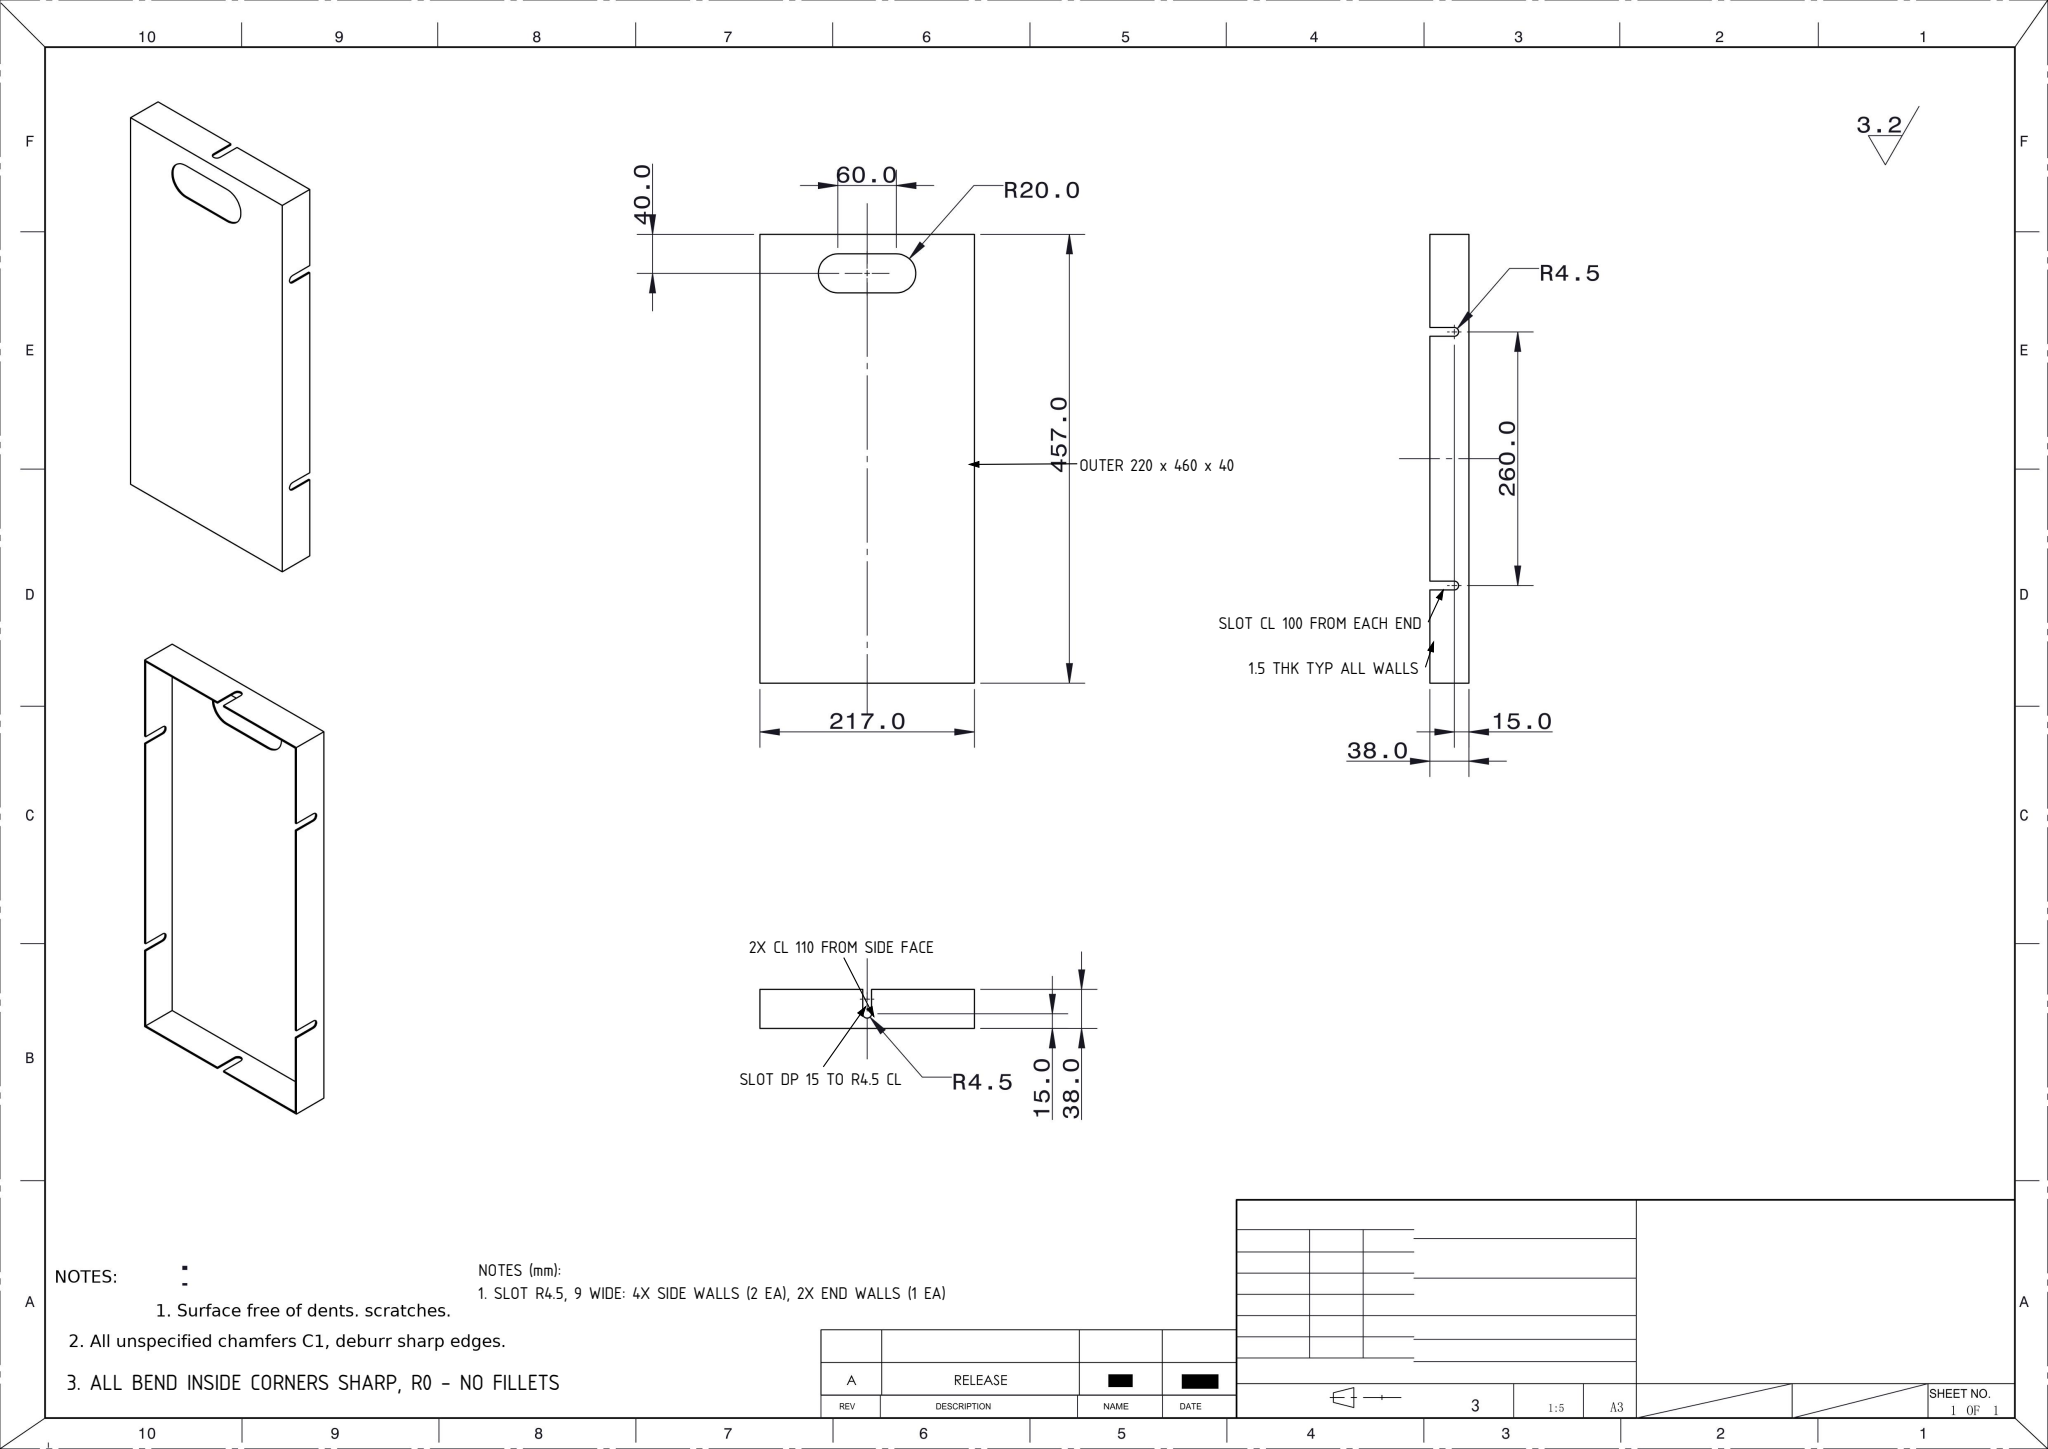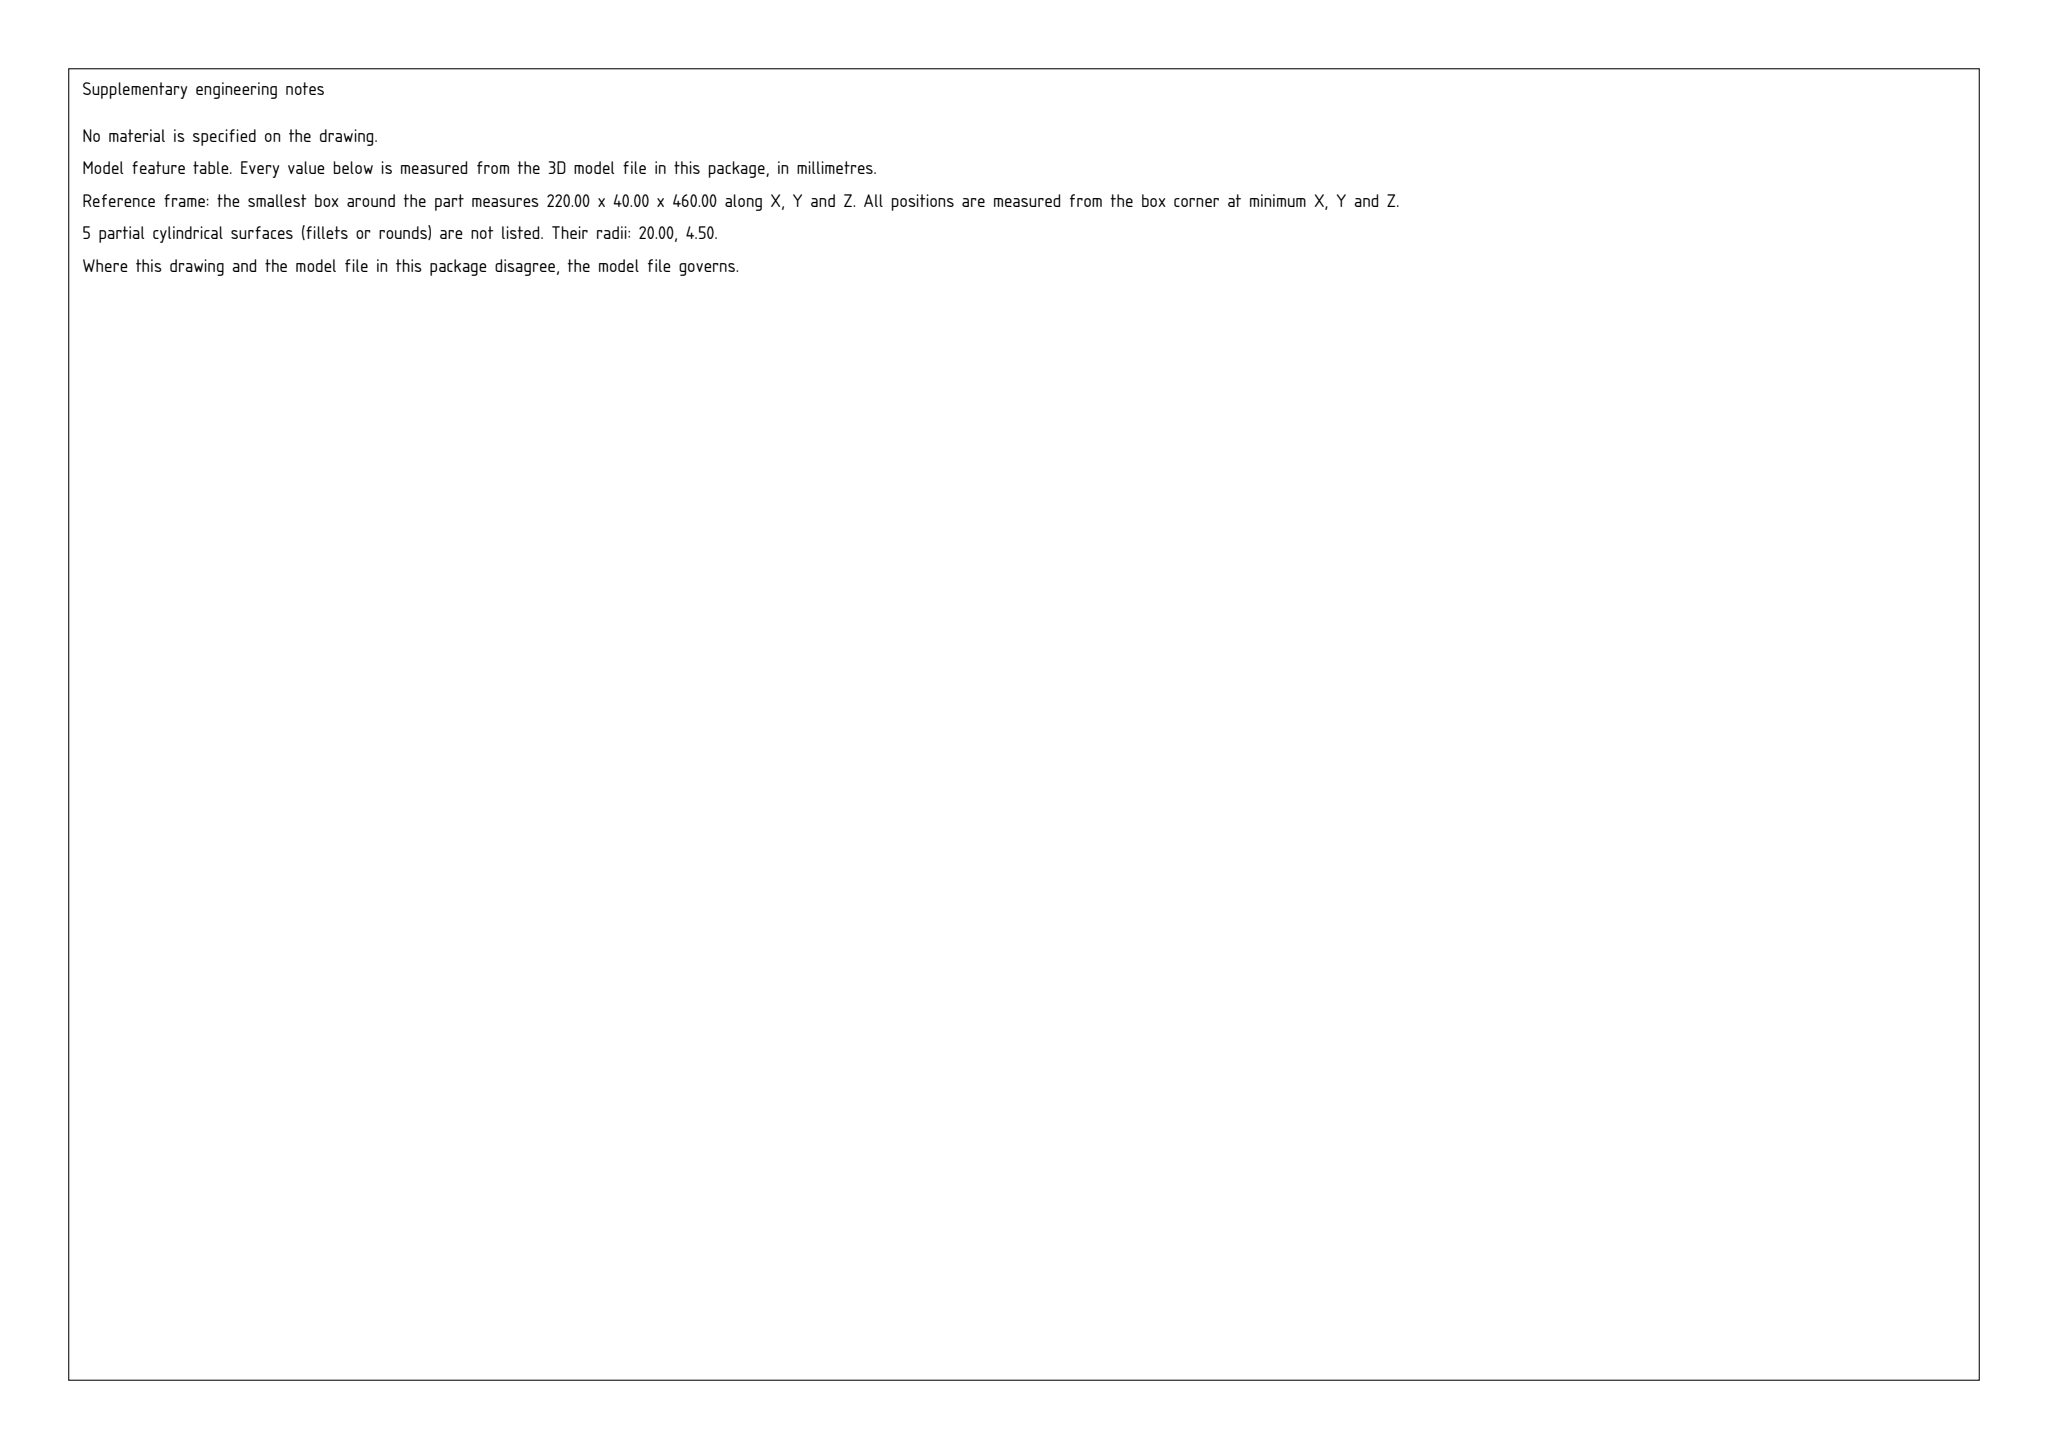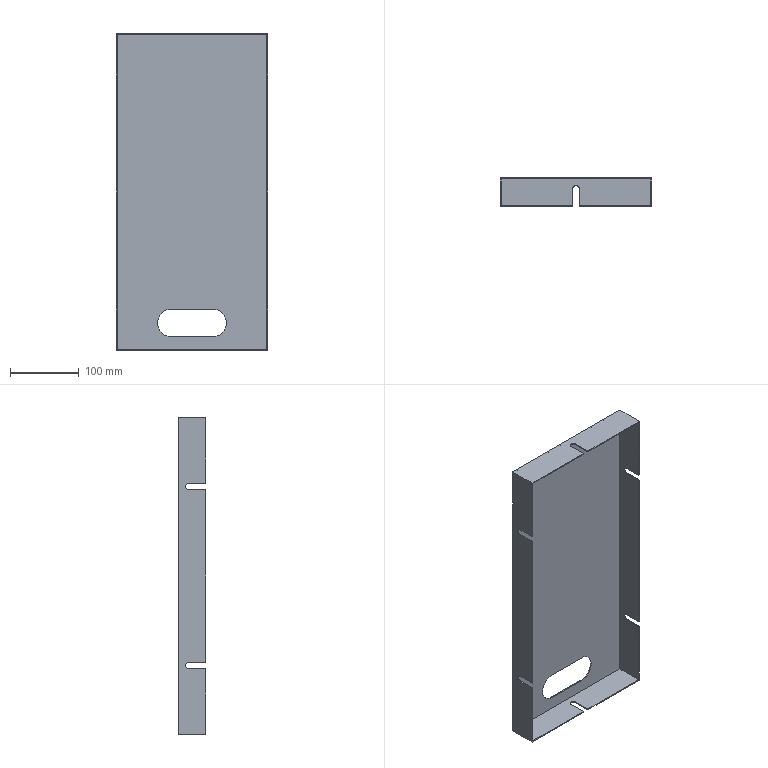Part | SolidWorks | mm | 1 solid | 38 faces | box 220 x 40 x 460 mm | volume 222197 mm3 | plane 30 | cylinder 8 | commonest cylinder face diameters 9 x6 40 x2
Drawing notes:
SHEET THK 1.5 TYP ALL WALLS, FORMED TRAY | from the solid: Planes x=0/1.5, x=218.5/220, z=0/1.5, z=458.5/460, y=38.5/40 give 1.5 wall
OVERALL OUTER ENVELOPE 220 x 460 x 40 (INNER 217 x 457) | from the solid: bbox_xyz 220.0 x 40.0 x 460.0; inner = 220-2x1.5, 460-2x1.5
ALL BEND INSIDE CORNERS SHARP, R0 - NO FILLETS | from the solid: fillet_radii: [] (empty), no cones/rounds at wall junctions
SLOT R4.5, 9 WIDE: 4X SIDE WALLS (2 EA), 2X END WALLS (1 EA) | from the solid: Ø9 x-axis cyl at z=100 (2) and z=360 (2); Ø9 z-axis cyl at x=110 (2)
SIDE WALL SLOT CL 100 FROM EACH END, 260 APART, TYP BOTH SIDES | from the solid: Ø9 x-axis cyl pos z=100 and z=360; 360-100=260; count 2 each
END WALL SLOT CL 110 FROM SIDE FACE, SYM ABOUT CL, 2X | from the solid: Ø9 z-axis cyl at x=110, count 2; bbox x=220 so 110 = CL
SLOT DEPTH 15.0 TO R4.5 CL FROM OPEN EDGE, THRU 1.5 WALL | from the solid: Ø9 cyl at y=25, wall y 0-40, length 1.5; 40-25=15
build123d program:
from build123d import *

# Parameters (mm, degrees)
SKETCH1_W           = 220
SKETCH1_H           = 460
BOSS_EXTRUDE1_DEPTH = 40
SHELL1_T            = -1.5
CUT_EXTRUDE1_DEPTH  = 1609.843
CUT_EXTRUDE2_DEPTH  = 1612.854
CUT_EXTRUDE3_DEPTH  = 502.897


with BuildPart() as part:
    # Sketch1 → Boss-Extrude1 (new body)
    with BuildSketch(Plane(origin=(0, 0, 0), x_dir=(1, 0, 0), z_dir=(0, 1, 0))):
        with Locations((-86.725, -1366.269)):
            Rectangle(SKETCH1_W, SKETCH1_H)
    extrude(amount=BOSS_EXTRUDE1_DEPTH)

    # Shell1
    shell1_openings = [part.faces().sort_by_distance(p)[0] for p in [
        (-86.725, 0, 1366.269),
    ]]
    offset(amount=SHELL1_T, openings=shell1_openings, kind=Kind.INTERSECTION)

    # Sketch2 → Cut-Extrude1 (cut, through all)
    with BuildSketch(Plane(origin=(0, 40, 0), x_dir=(1, 0, 0), z_dir=(0, 1, 0))):
        with BuildLine():
            Line((-56.725, -1196.269), (-116.725, -1196.269))
            ThreePointArc((-116.725, -1196.269), (-136.725, -1176.269), (-116.725, -1156.269))
            Line((-116.725, -1156.269), (-56.725, -1156.269))
            ThreePointArc((-56.725, -1156.269), (-36.725, -1176.269), (-56.725, -1196.269))
        make_face()
    extrude(amount=-CUT_EXTRUDE1_DEPTH, mode=Mode.SUBTRACT)

    # Sketch3 → Cut-Extrude2 (cut, through all)
    with BuildSketch(Plane(origin=(23.275, 0, 0), x_dir=(0, 0, -1), z_dir=(1, 0, 0))):
        with BuildLine():
            Line((-1500.769, -5), (-1500.769, 25))
            ThreePointArc((-1500.769, 25), (-1496.269, 29.5), (-1491.769, 25))
            Line((-1491.769, 25), (-1491.769, -5))
            ThreePointArc((-1491.769, -5), (-1496.269, -9.5), (-1500.769, -5))
        make_face()
        with BuildLine():
            Line((-1231.769, -5), (-1231.769, 25))
            ThreePointArc((-1231.769, 25), (-1236.269, 29.5), (-1240.769, 25))
            Line((-1240.769, 25), (-1240.769, -5))
            ThreePointArc((-1240.769, -5), (-1236.269, -9.5), (-1231.769, -5))
        make_face()
    extrude(amount=-CUT_EXTRUDE2_DEPTH, mode=Mode.SUBTRACT)

    # Sketch4 → Cut-Extrude3 (cut, through all)
    with BuildSketch(Plane.XY.offset(1596.269)):
        with BuildLine():
            Line((-91.225, -5), (-91.225, 25))
            ThreePointArc((-91.225, 25), (-86.725, 29.5), (-82.225, 25))
            Line((-82.225, 25), (-82.225, -5))
            ThreePointArc((-82.225, -5), (-86.725, -9.5), (-91.225, -5))
        make_face()
    extrude(amount=-CUT_EXTRUDE3_DEPTH, mode=Mode.SUBTRACT)


solid = part.part